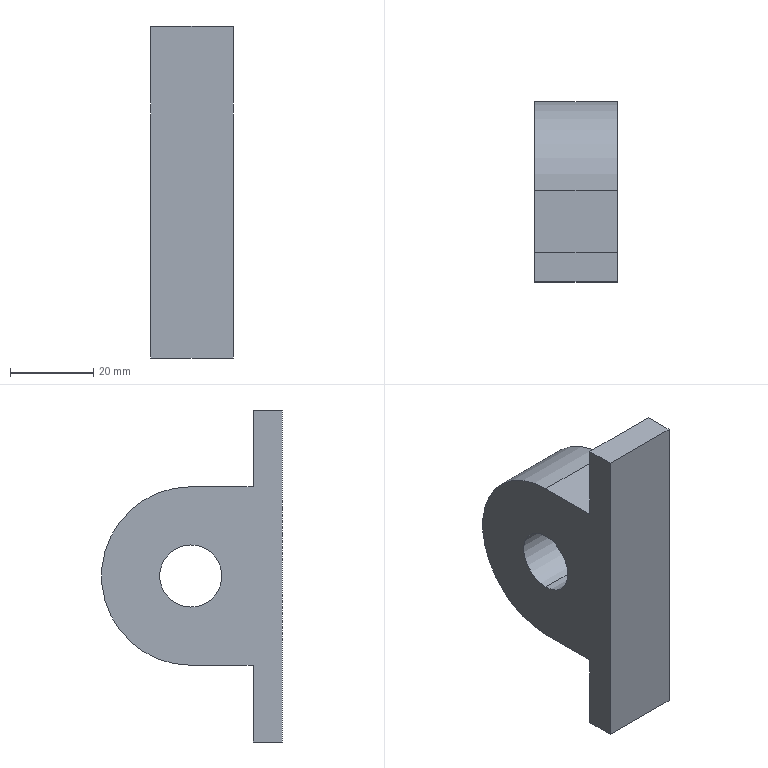Component | SolidWorks | p002-2 | 1 solid | 12 faces | box 20 x 43.5 x 80 mm | volume 35088 mm3 | plane 9 | cylinder 3 | commonest cylinder face diameters 15 x2 43 x1
build123d program:
from build123d import *

# Parameters (mm, degrees)
SKETCH1_R      = 7.5
EXTRUDE1_DEPTH = 20


with BuildPart() as part:
    # Sketch1 → Extrude1 (new body)
    with BuildSketch(Plane.XY):
        with BuildLine():
            Line((-40, 3.5), (-21.5, 3.5))
            Line((-21.5, 3.5), (-21.5, 18.5))
            ThreePointArc((-21.5, 18.5), (0, 40), (21.5, 18.5))
            Line((21.5, 18.5), (21.5, 3.5))
            Line((21.5, 3.5), (40, 3.5))
            Line((40, 3.5), (40, -3.5))
            Line((40, -3.5), (-40, -3.5))
            Line((-40, -3.5), (-40, 3.5))
        make_face()
        with Locations((0, 18.5)):
            Circle(SKETCH1_R, mode=Mode.SUBTRACT)
    extrude(amount=EXTRUDE1_DEPTH)


solid = part.part

# Placed as in the assembly
solid = solid.moved(Location((170.216, 157.483, 58.736), (0, 90, 0)))
STEP:
#1=COLOUR_RGB('',0.7922,0.8196,0.9333);
#2=FILL_AREA_STYLE_COLOUR('',#1);
#3=FILL_AREA_STYLE('',(#2));
#4=SURFACE_STYLE_FILL_AREA(#3);
#5=SURFACE_SIDE_STYLE('',(#4));
#6=SURFACE_STYLE_USAGE(.BOTH.,#5);
#7=PRESENTATION_STYLE_ASSIGNMENT((#6));
#8=CARTESIAN_POINT('',(7.489,6.928,2.608));
#9=VERTEX_POINT('',#8);
#10=CARTESIAN_POINT('',(7.489,6.928,2.017));
#11=VERTEX_POINT('',#10);
#12=CARTESIAN_POINT('',(7.489,6.928,2.312));
#13=DIRECTION('',(1.,0.,0.));
#14=DIRECTION('',(0.,0.,-1.));
#15=AXIS2_PLACEMENT_3D('',#12,#13,#14);
#16=CIRCLE('',#15,0.2953);
#17=EDGE_CURVE('',#9,#11,#16,.T.);
#18=ORIENTED_EDGE('',*,*,#17,.T.);
#19=CARTESIAN_POINT('',(6.701,6.928,2.017));
#20=VERTEX_POINT('',#19);
#21=CARTESIAN_POINT('',(7.489,6.928,2.017));
#22=DIRECTION('',(-1.,-0.,-0.));
#23=VECTOR('',#22,39.37);
#24=LINE('',#21,#23);
#25=EDGE_CURVE('',#11,#20,#24,.T.);
#26=ORIENTED_EDGE('',*,*,#25,.T.);
#27=CARTESIAN_POINT('',(6.701,6.928,2.608));
#28=VERTEX_POINT('',#27);
#29=CARTESIAN_POINT('',(6.701,6.928,2.312));
#30=DIRECTION('',(1.,0.,0.));
#31=DIRECTION('',(0.,0.,-1.));
#32=AXIS2_PLACEMENT_3D('',#29,#30,#31);
#33=CIRCLE('',#32,0.2953);
#34=EDGE_CURVE('',#28,#20,#33,.T.);
#35=ORIENTED_EDGE('',*,*,#34,.F.);
#36=CARTESIAN_POINT('',(7.489,6.928,2.608));
#37=DIRECTION('',(-1.,-0.,-0.));
#38=VECTOR('',#37,39.37);
#39=LINE('',#36,#38);
#40=EDGE_CURVE('',#9,#28,#39,.T.);
#41=ORIENTED_EDGE('',*,*,#40,.F.);
#42=EDGE_LOOP('',(#18,#26,#35,#41));
#43=FACE_OUTER_BOUND('',#42,.T.);
#44=CARTESIAN_POINT('',(7.489,6.928,2.312));
#45=DIRECTION('',(-1.,-0.,-0.));
#46=DIRECTION('',(0.,0.,1.));
#47=AXIS2_PLACEMENT_3D('',#44,#45,#46);
#48=CYLINDRICAL_SURFACE('',#47,0.2953);
#49=ADVANCED_FACE('',(#43),#48,.F.);
#50=CARTESIAN_POINT('',(7.489,6.338,3.887));
#51=VERTEX_POINT('',#50);
#52=CARTESIAN_POINT('',(7.489,6.062,3.887));
#53=VERTEX_POINT('',#52);
#54=CARTESIAN_POINT('',(7.489,6.338,3.887));
#55=DIRECTION('',(0.,-1.,0.));
#56=VECTOR('',#55,39.37);
#57=LINE('',#54,#56);
#58=EDGE_CURVE('',#51,#53,#57,.T.);
#59=ORIENTED_EDGE('',*,*,#58,.T.);
#60=CARTESIAN_POINT('',(7.489,6.062,0.7377));
#61=VERTEX_POINT('',#60);
#62=CARTESIAN_POINT('',(7.489,6.062,3.887));
#63=DIRECTION('',(0.,-0.,-1.));
#64=VECTOR('',#63,39.37);
#65=LINE('',#62,#64);
#66=EDGE_CURVE('',#53,#61,#65,.T.);
#67=ORIENTED_EDGE('',*,*,#66,.T.);
#68=CARTESIAN_POINT('',(7.489,6.338,0.7377));
#69=VERTEX_POINT('',#68);
#70=CARTESIAN_POINT('',(7.489,6.338,0.7377));
#71=DIRECTION('',(-0.,1.,-0.));
#72=VECTOR('',#71,39.37);
#73=LINE('',#70,#72);
#74=EDGE_CURVE('',#61,#69,#73,.T.);
#75=ORIENTED_EDGE('',*,*,#74,.T.);
#76=CARTESIAN_POINT('',(7.489,6.338,1.466));
#77=VERTEX_POINT('',#76);
#78=CARTESIAN_POINT('',(7.489,6.338,1.466));
#79=DIRECTION('',(-0.,0.,1.));
#80=VECTOR('',#79,39.37);
#81=LINE('',#78,#80);
#82=EDGE_CURVE('',#69,#77,#81,.T.);
#83=ORIENTED_EDGE('',*,*,#82,.T.);
#84=CARTESIAN_POINT('',(7.489,6.928,1.466));
#85=VERTEX_POINT('',#84);
#86=CARTESIAN_POINT('',(7.489,6.928,1.466));
#87=DIRECTION('',(-0.,1.,0.));
#88=VECTOR('',#87,39.37);
#89=LINE('',#86,#88);
#90=EDGE_CURVE('',#77,#85,#89,.T.);
#91=ORIENTED_EDGE('',*,*,#90,.T.);
#92=CARTESIAN_POINT('',(7.489,6.928,3.159));
#93=VERTEX_POINT('',#92);
#94=CARTESIAN_POINT('',(7.489,6.928,2.312));
#95=DIRECTION('',(1.,0.,0.));
#96=DIRECTION('',(0.,0.,-1.));
#97=AXIS2_PLACEMENT_3D('',#94,#95,#96);
#98=CIRCLE('',#97,0.8465);
#99=EDGE_CURVE('',#85,#93,#98,.T.);
#100=ORIENTED_EDGE('',*,*,#99,.T.);
#101=CARTESIAN_POINT('',(7.489,6.338,3.159));
#102=VERTEX_POINT('',#101);
#103=CARTESIAN_POINT('',(7.489,6.928,3.159));
#104=DIRECTION('',(0.,-1.,0.));
#105=VECTOR('',#104,39.37);
#106=LINE('',#103,#105);
#107=EDGE_CURVE('',#93,#102,#106,.T.);
#108=ORIENTED_EDGE('',*,*,#107,.T.);
#109=CARTESIAN_POINT('',(7.489,6.338,3.887));
#110=DIRECTION('',(-0.,0.,1.));
#111=VECTOR('',#110,39.37);
#112=LINE('',#109,#111);
#113=EDGE_CURVE('',#102,#51,#112,.T.);
#114=ORIENTED_EDGE('',*,*,#113,.T.);
#115=EDGE_LOOP('',(#59,#67,#75,#83,#91,#100,#108,#114));
#116=FACE_OUTER_BOUND('',#115,.T.);
#117=ORIENTED_EDGE('',*,*,#17,.F.);
#118=CARTESIAN_POINT('',(7.489,6.928,2.312));
#119=DIRECTION('',(1.,0.,0.));
#120=DIRECTION('',(0.,0.,-1.));
#121=AXIS2_PLACEMENT_3D('',#118,#119,#120);
#122=CIRCLE('',#121,0.2953);
#123=EDGE_CURVE('',#11,#9,#122,.T.);
#124=ORIENTED_EDGE('',*,*,#123,.F.);
#125=EDGE_LOOP('',(#117,#124));
#126=FACE_BOUND('',#125,.T.);
#127=CARTESIAN_POINT('',(7.489,6.928,2.312));
#128=DIRECTION('',(1.,0.,0.));
#129=DIRECTION('',(0.,-0.,-1.));
#130=AXIS2_PLACEMENT_3D('',#127,#128,#129);
#131=PLANE('',#130);
#132=ADVANCED_FACE('',(#116,#126),#131,.T.);
#133=CARTESIAN_POINT('',(6.701,6.338,3.887));
#134=VERTEX_POINT('',#133);
#135=CARTESIAN_POINT('',(6.701,6.062,3.887));
#136=VERTEX_POINT('',#135);
#137=CARTESIAN_POINT('',(6.701,6.338,3.887));
#138=DIRECTION('',(0.,-1.,0.));
#139=VECTOR('',#138,39.37);
#140=LINE('',#137,#139);
#141=EDGE_CURVE('',#134,#136,#140,.T.);
#142=ORIENTED_EDGE('',*,*,#141,.F.);
#143=CARTESIAN_POINT('',(6.701,6.338,3.159));
#144=VERTEX_POINT('',#143);
#145=CARTESIAN_POINT('',(6.701,6.338,3.887));
#146=DIRECTION('',(-0.,0.,1.));
#147=VECTOR('',#146,39.37);
#148=LINE('',#145,#147);
#149=EDGE_CURVE('',#144,#134,#148,.T.);
#150=ORIENTED_EDGE('',*,*,#149,.F.);
#151=CARTESIAN_POINT('',(6.701,6.928,3.159));
#152=VERTEX_POINT('',#151);
#153=CARTESIAN_POINT('',(6.701,6.928,3.159));
#154=DIRECTION('',(0.,-1.,0.));
#155=VECTOR('',#154,39.37);
#156=LINE('',#153,#155);
#157=EDGE_CURVE('',#152,#144,#156,.T.);
#158=ORIENTED_EDGE('',*,*,#157,.F.);
#159=CARTESIAN_POINT('',(6.701,6.928,1.466));
#160=VERTEX_POINT('',#159);
#161=CARTESIAN_POINT('',(6.701,6.928,2.312));
#162=DIRECTION('',(1.,0.,0.));
#163=DIRECTION('',(0.,0.,-1.));
#164=AXIS2_PLACEMENT_3D('',#161,#162,#163);
#165=CIRCLE('',#164,0.8465);
#166=EDGE_CURVE('',#160,#152,#165,.T.);
#167=ORIENTED_EDGE('',*,*,#166,.F.);
#168=CARTESIAN_POINT('',(6.701,6.338,1.466));
#169=VERTEX_POINT('',#168);
#170=CARTESIAN_POINT('',(6.701,6.928,1.466));
#171=DIRECTION('',(-0.,1.,0.));
#172=VECTOR('',#171,39.37);
#173=LINE('',#170,#172);
#174=EDGE_CURVE('',#169,#160,#173,.T.);
#175=ORIENTED_EDGE('',*,*,#174,.F.);
#176=CARTESIAN_POINT('',(6.701,6.338,0.7377));
#177=VERTEX_POINT('',#176);
#178=CARTESIAN_POINT('',(6.701,6.338,1.466));
#179=DIRECTION('',(-0.,0.,1.));
#180=VECTOR('',#179,39.37);
#181=LINE('',#178,#180);
#182=EDGE_CURVE('',#177,#169,#181,.T.);
#183=ORIENTED_EDGE('',*,*,#182,.F.);
#184=CARTESIAN_POINT('',(6.701,6.062,0.7377));
#185=VERTEX_POINT('',#184);
#186=CARTESIAN_POINT('',(6.701,6.338,0.7377));
#187=DIRECTION('',(-0.,1.,-0.));
#188=VECTOR('',#187,39.37);
#189=LINE('',#186,#188);
#190=EDGE_CURVE('',#185,#177,#189,.T.);
#191=ORIENTED_EDGE('',*,*,#190,.F.);
#192=CARTESIAN_POINT('',(6.701,6.062,3.887));
#193=DIRECTION('',(0.,-0.,-1.));
#194=VECTOR('',#193,39.37);
#195=LINE('',#192,#194);
#196=EDGE_CURVE('',#136,#185,#195,.T.);
#197=ORIENTED_EDGE('',*,*,#196,.F.);
#198=EDGE_LOOP('',(#142,#150,#158,#167,#175,#183,#191,#197));
#199=FACE_OUTER_BOUND('',#198,.T.);
#200=ORIENTED_EDGE('',*,*,#34,.T.);
#201=CARTESIAN_POINT('',(6.701,6.928,2.312));
#202=DIRECTION('',(1.,0.,0.));
#203=DIRECTION('',(0.,0.,-1.));
#204=AXIS2_PLACEMENT_3D('',#201,#202,#203);
#205=CIRCLE('',#204,0.2953);
#206=EDGE_CURVE('',#20,#28,#205,.T.);
#207=ORIENTED_EDGE('',*,*,#206,.T.);
#208=EDGE_LOOP('',(#200,#207));
#209=FACE_BOUND('',#208,.T.);
#210=CARTESIAN_POINT('',(6.701,6.928,2.312));
#211=DIRECTION('',(1.,0.,0.));
#212=DIRECTION('',(0.,-0.,-1.));
#213=AXIS2_PLACEMENT_3D('',#210,#211,#212);
#214=PLANE('',#213);
#215=ADVANCED_FACE('',(#199,#209),#214,.F.);
#216=ORIENTED_EDGE('',*,*,#141,.T.);
#217=CARTESIAN_POINT('',(7.489,6.062,3.887));
#218=DIRECTION('',(-1.,-0.,-0.));
#219=VECTOR('',#218,39.37);
#220=LINE('',#217,#219);
#221=EDGE_CURVE('',#53,#136,#220,.T.);
#222=ORIENTED_EDGE('',*,*,#221,.F.);
#223=ORIENTED_EDGE('',*,*,#58,.F.);
#224=CARTESIAN_POINT('',(7.489,6.338,3.887));
#225=DIRECTION('',(-1.,-0.,-0.));
#226=VECTOR('',#225,39.37);
#227=LINE('',#224,#226);
#228=EDGE_CURVE('',#51,#134,#227,.T.);
#229=ORIENTED_EDGE('',*,*,#228,.T.);
#230=EDGE_LOOP('',(#216,#222,#223,#229));
#231=FACE_OUTER_BOUND('',#230,.T.);
#232=CARTESIAN_POINT('',(7.489,6.338,3.887));
#233=DIRECTION('',(0.,-0.,-1.));
#234=DIRECTION('',(-1.,-0.,-0.));
#235=AXIS2_PLACEMENT_3D('',#232,#233,#234);
#236=PLANE('',#235);
#237=ADVANCED_FACE('',(#231),#236,.F.);
#238=ORIENTED_EDGE('',*,*,#196,.T.);
#239=CARTESIAN_POINT('',(7.489,6.062,0.7377));
#240=DIRECTION('',(-1.,-0.,-0.));
#241=VECTOR('',#240,39.37);
#242=LINE('',#239,#241);
#243=EDGE_CURVE('',#61,#185,#242,.T.);
#244=ORIENTED_EDGE('',*,*,#243,.F.);
#245=ORIENTED_EDGE('',*,*,#66,.F.);
#246=ORIENTED_EDGE('',*,*,#221,.T.);
#247=EDGE_LOOP('',(#238,#244,#245,#246));
#248=FACE_OUTER_BOUND('',#247,.T.);
#249=CARTESIAN_POINT('',(7.489,6.062,3.887));
#250=DIRECTION('',(-0.,1.,-0.));
#251=DIRECTION('',(1.,0.,0.));
#252=AXIS2_PLACEMENT_3D('',#249,#250,#251);
#253=PLANE('',#252);
#254=ADVANCED_FACE('',(#248),#253,.F.);
#255=ORIENTED_EDGE('',*,*,#190,.T.);
#256=CARTESIAN_POINT('',(7.489,6.338,0.7377));
#257=DIRECTION('',(-1.,-0.,-0.));
#258=VECTOR('',#257,39.37);
#259=LINE('',#256,#258);
#260=EDGE_CURVE('',#69,#177,#259,.T.);
#261=ORIENTED_EDGE('',*,*,#260,.F.);
#262=ORIENTED_EDGE('',*,*,#74,.F.);
#263=ORIENTED_EDGE('',*,*,#243,.T.);
#264=EDGE_LOOP('',(#255,#261,#262,#263));
#265=FACE_OUTER_BOUND('',#264,.T.);
#266=CARTESIAN_POINT('',(7.489,6.338,0.7377));
#267=DIRECTION('',(-0.,0.,1.));
#268=DIRECTION('',(1.,0.,0.));
#269=AXIS2_PLACEMENT_3D('',#266,#267,#268);
#270=PLANE('',#269);
#271=ADVANCED_FACE('',(#265),#270,.F.);
#272=ORIENTED_EDGE('',*,*,#182,.T.);
#273=CARTESIAN_POINT('',(7.489,6.338,1.466));
#274=DIRECTION('',(-1.,-0.,-0.));
#275=VECTOR('',#274,39.37);
#276=LINE('',#273,#275);
#277=EDGE_CURVE('',#77,#169,#276,.T.);
#278=ORIENTED_EDGE('',*,*,#277,.F.);
#279=ORIENTED_EDGE('',*,*,#82,.F.);
#280=ORIENTED_EDGE('',*,*,#260,.T.);
#281=EDGE_LOOP('',(#272,#278,#279,#280));
#282=FACE_OUTER_BOUND('',#281,.T.);
#283=CARTESIAN_POINT('',(7.489,6.338,1.466));
#284=DIRECTION('',(0.,-1.,0.));
#285=DIRECTION('',(-1.,-0.,-0.));
#286=AXIS2_PLACEMENT_3D('',#283,#284,#285);
#287=PLANE('',#286);
#288=ADVANCED_FACE('',(#282),#287,.F.);
#289=ORIENTED_EDGE('',*,*,#174,.T.);
#290=CARTESIAN_POINT('',(7.489,6.928,1.466));
#291=DIRECTION('',(-1.,-0.,-0.));
#292=VECTOR('',#291,39.37);
#293=LINE('',#290,#292);
#294=EDGE_CURVE('',#85,#160,#293,.T.);
#295=ORIENTED_EDGE('',*,*,#294,.F.);
#296=ORIENTED_EDGE('',*,*,#90,.F.);
#297=ORIENTED_EDGE('',*,*,#277,.T.);
#298=EDGE_LOOP('',(#289,#295,#296,#297));
#299=FACE_OUTER_BOUND('',#298,.T.);
#300=CARTESIAN_POINT('',(7.489,6.928,1.466));
#301=DIRECTION('',(-0.,-0.,1.));
#302=DIRECTION('',(0.,-1.,-0.));
#303=AXIS2_PLACEMENT_3D('',#300,#301,#302);
#304=PLANE('',#303);
#305=ADVANCED_FACE('',(#299),#304,.F.);
#306=ORIENTED_EDGE('',*,*,#166,.T.);
#307=CARTESIAN_POINT('',(7.489,6.928,3.159));
#308=DIRECTION('',(-1.,-0.,-0.));
#309=VECTOR('',#308,39.37);
#310=LINE('',#307,#309);
#311=EDGE_CURVE('',#93,#152,#310,.T.);
#312=ORIENTED_EDGE('',*,*,#311,.F.);
#313=ORIENTED_EDGE('',*,*,#99,.F.);
#314=ORIENTED_EDGE('',*,*,#294,.T.);
#315=EDGE_LOOP('',(#306,#312,#313,#314));
#316=FACE_OUTER_BOUND('',#315,.T.);
#317=CARTESIAN_POINT('',(7.489,6.928,2.312));
#318=DIRECTION('',(-1.,-0.,-0.));
#319=DIRECTION('',(0.,0.,1.));
#320=AXIS2_PLACEMENT_3D('',#317,#318,#319);
#321=CYLINDRICAL_SURFACE('',#320,0.8465);
#322=ADVANCED_FACE('',(#316),#321,.T.);
#323=ORIENTED_EDGE('',*,*,#157,.T.);
#324=CARTESIAN_POINT('',(7.489,6.338,3.159));
#325=DIRECTION('',(-1.,-0.,-0.));
#326=VECTOR('',#325,39.37);
#327=LINE('',#324,#326);
#328=EDGE_CURVE('',#102,#144,#327,.T.);
#329=ORIENTED_EDGE('',*,*,#328,.F.);
#330=ORIENTED_EDGE('',*,*,#107,.F.);
#331=ORIENTED_EDGE('',*,*,#311,.T.);
#332=EDGE_LOOP('',(#323,#329,#330,#331));
#333=FACE_OUTER_BOUND('',#332,.T.);
#334=CARTESIAN_POINT('',(7.489,6.928,3.159));
#335=DIRECTION('',(0.,-0.,-1.));
#336=DIRECTION('',(-0.,1.,-0.));
#337=AXIS2_PLACEMENT_3D('',#334,#335,#336);
#338=PLANE('',#337);
#339=ADVANCED_FACE('',(#333),#338,.F.);
#340=ORIENTED_EDGE('',*,*,#149,.T.);
#341=ORIENTED_EDGE('',*,*,#228,.F.);
#342=ORIENTED_EDGE('',*,*,#113,.F.);
#343=ORIENTED_EDGE('',*,*,#328,.T.);
#344=EDGE_LOOP('',(#340,#341,#342,#343));
#345=FACE_OUTER_BOUND('',#344,.T.);
#346=CARTESIAN_POINT('',(7.489,6.338,3.887));
#347=DIRECTION('',(0.,-1.,0.));
#348=DIRECTION('',(-1.,-0.,-0.));
#349=AXIS2_PLACEMENT_3D('',#346,#347,#348);
#350=PLANE('',#349);
#351=ADVANCED_FACE('',(#345),#350,.F.);
#352=ORIENTED_EDGE('',*,*,#25,.F.);
#353=ORIENTED_EDGE('',*,*,#123,.T.);
#354=ORIENTED_EDGE('',*,*,#40,.T.);
#355=ORIENTED_EDGE('',*,*,#206,.F.);
#356=EDGE_LOOP('',(#352,#353,#354,#355));
#357=FACE_OUTER_BOUND('',#356,.T.);
#358=CARTESIAN_POINT('',(7.489,6.928,2.312));
#359=DIRECTION('',(-1.,-0.,-0.));
#360=DIRECTION('',(0.,0.,1.));
#361=AXIS2_PLACEMENT_3D('',#358,#359,#360);
#362=CYLINDRICAL_SURFACE('',#361,0.2953);
#363=ADVANCED_FACE('',(#357),#362,.F.);
#364=CLOSED_SHELL('',(#49,#132,#215,#237,#254,#271,#288,#305,#322,#339,#351,#363));
#365=MANIFOLD_SOLID_BREP('',#364);
#366=STYLED_ITEM('',(#7),#365);
#367=PRESENTATION_LAYER_ASSIGNMENT('','',(#366));
#368=CARTESIAN_POINT('',(0.,0.,0.));
#369=DIRECTION('',(0.,0.,1.));
#370=DIRECTION('',(1.,0.,0.));
#371=AXIS2_PLACEMENT_3D('',#368,#369,#370);
#372=(LENGTH_UNIT()NAMED_UNIT(*)SI_UNIT($,.METRE.));
#373=LENGTH_MEASURE_WITH_UNIT(LENGTH_MEASURE(0.0254),#372);
#374=DIMENSIONAL_EXPONENTS(1.,0.,0.,0.,0.,0.,0.);
#375=(CONVERSION_BASED_UNIT('',#373)LENGTH_UNIT()NAMED_UNIT(#374));
#376=UNCERTAINTY_MEASURE_WITH_UNIT(LENGTH_MEASURE(0.00001),#375,'','');
#377=(NAMED_UNIT(*)PLANE_ANGLE_UNIT()SI_UNIT($,.RADIAN.));
#378=(NAMED_UNIT(*)SI_UNIT($,.STERADIAN.)SOLID_ANGLE_UNIT());
#379=(GEOMETRIC_REPRESENTATION_CONTEXT(3)GLOBAL_UNCERTAINTY_ASSIGNED_CONTEXT((#376))GLOBAL_UNIT_ASSIGNED_CONTEXT((#375,#377,#378))REPRESENTATION_CONTEXT('',''));
#380=ADVANCED_BREP_SHAPE_REPRESENTATION('',(#365,#371),#379);
#381=(LENGTH_UNIT()NAMED_UNIT(*)SI_UNIT($,.METRE.));
#382=LENGTH_MEASURE_WITH_UNIT(LENGTH_MEASURE(0.0254),#381);
#383=DIMENSIONAL_EXPONENTS(1.,0.,0.,0.,0.,0.,0.);
#384=(CONVERSION_BASED_UNIT('',#382)LENGTH_UNIT()NAMED_UNIT(#383));
#385=UNCERTAINTY_MEASURE_WITH_UNIT(LENGTH_MEASURE(0.00001),#384,'','');
#386=(NAMED_UNIT(*)PLANE_ANGLE_UNIT()SI_UNIT($,.RADIAN.));
#387=(NAMED_UNIT(*)SI_UNIT($,.STERADIAN.)SOLID_ANGLE_UNIT());
#388=(GEOMETRIC_REPRESENTATION_CONTEXT(3)GLOBAL_UNCERTAINTY_ASSIGNED_CONTEXT((#385))GLOBAL_UNIT_ASSIGNED_CONTEXT((#384,#386,#387))REPRESENTATION_CONTEXT('',''));
#389=MECHANICAL_DESIGN_GEOMETRIC_PRESENTATION_REPRESENTATION('',(#366),#388);